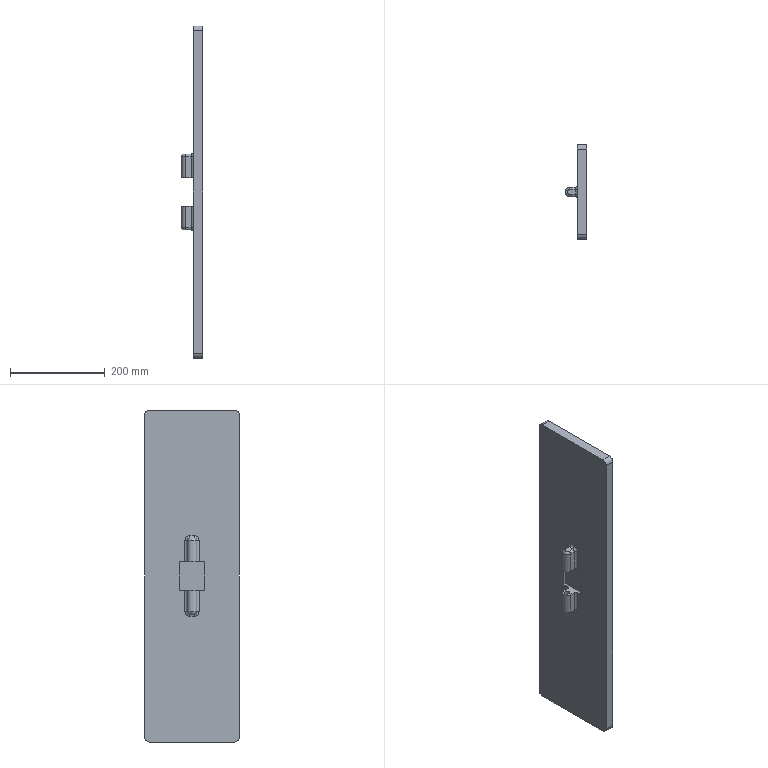Component | NX | MODEL1 | 1 solid | 53 faces | volume 2601003 mm3 | plane 29 | cylinder 18 | torus 4 | spline 2 | commonest cylinder face diameters 10 x10 20 x6 11 x2